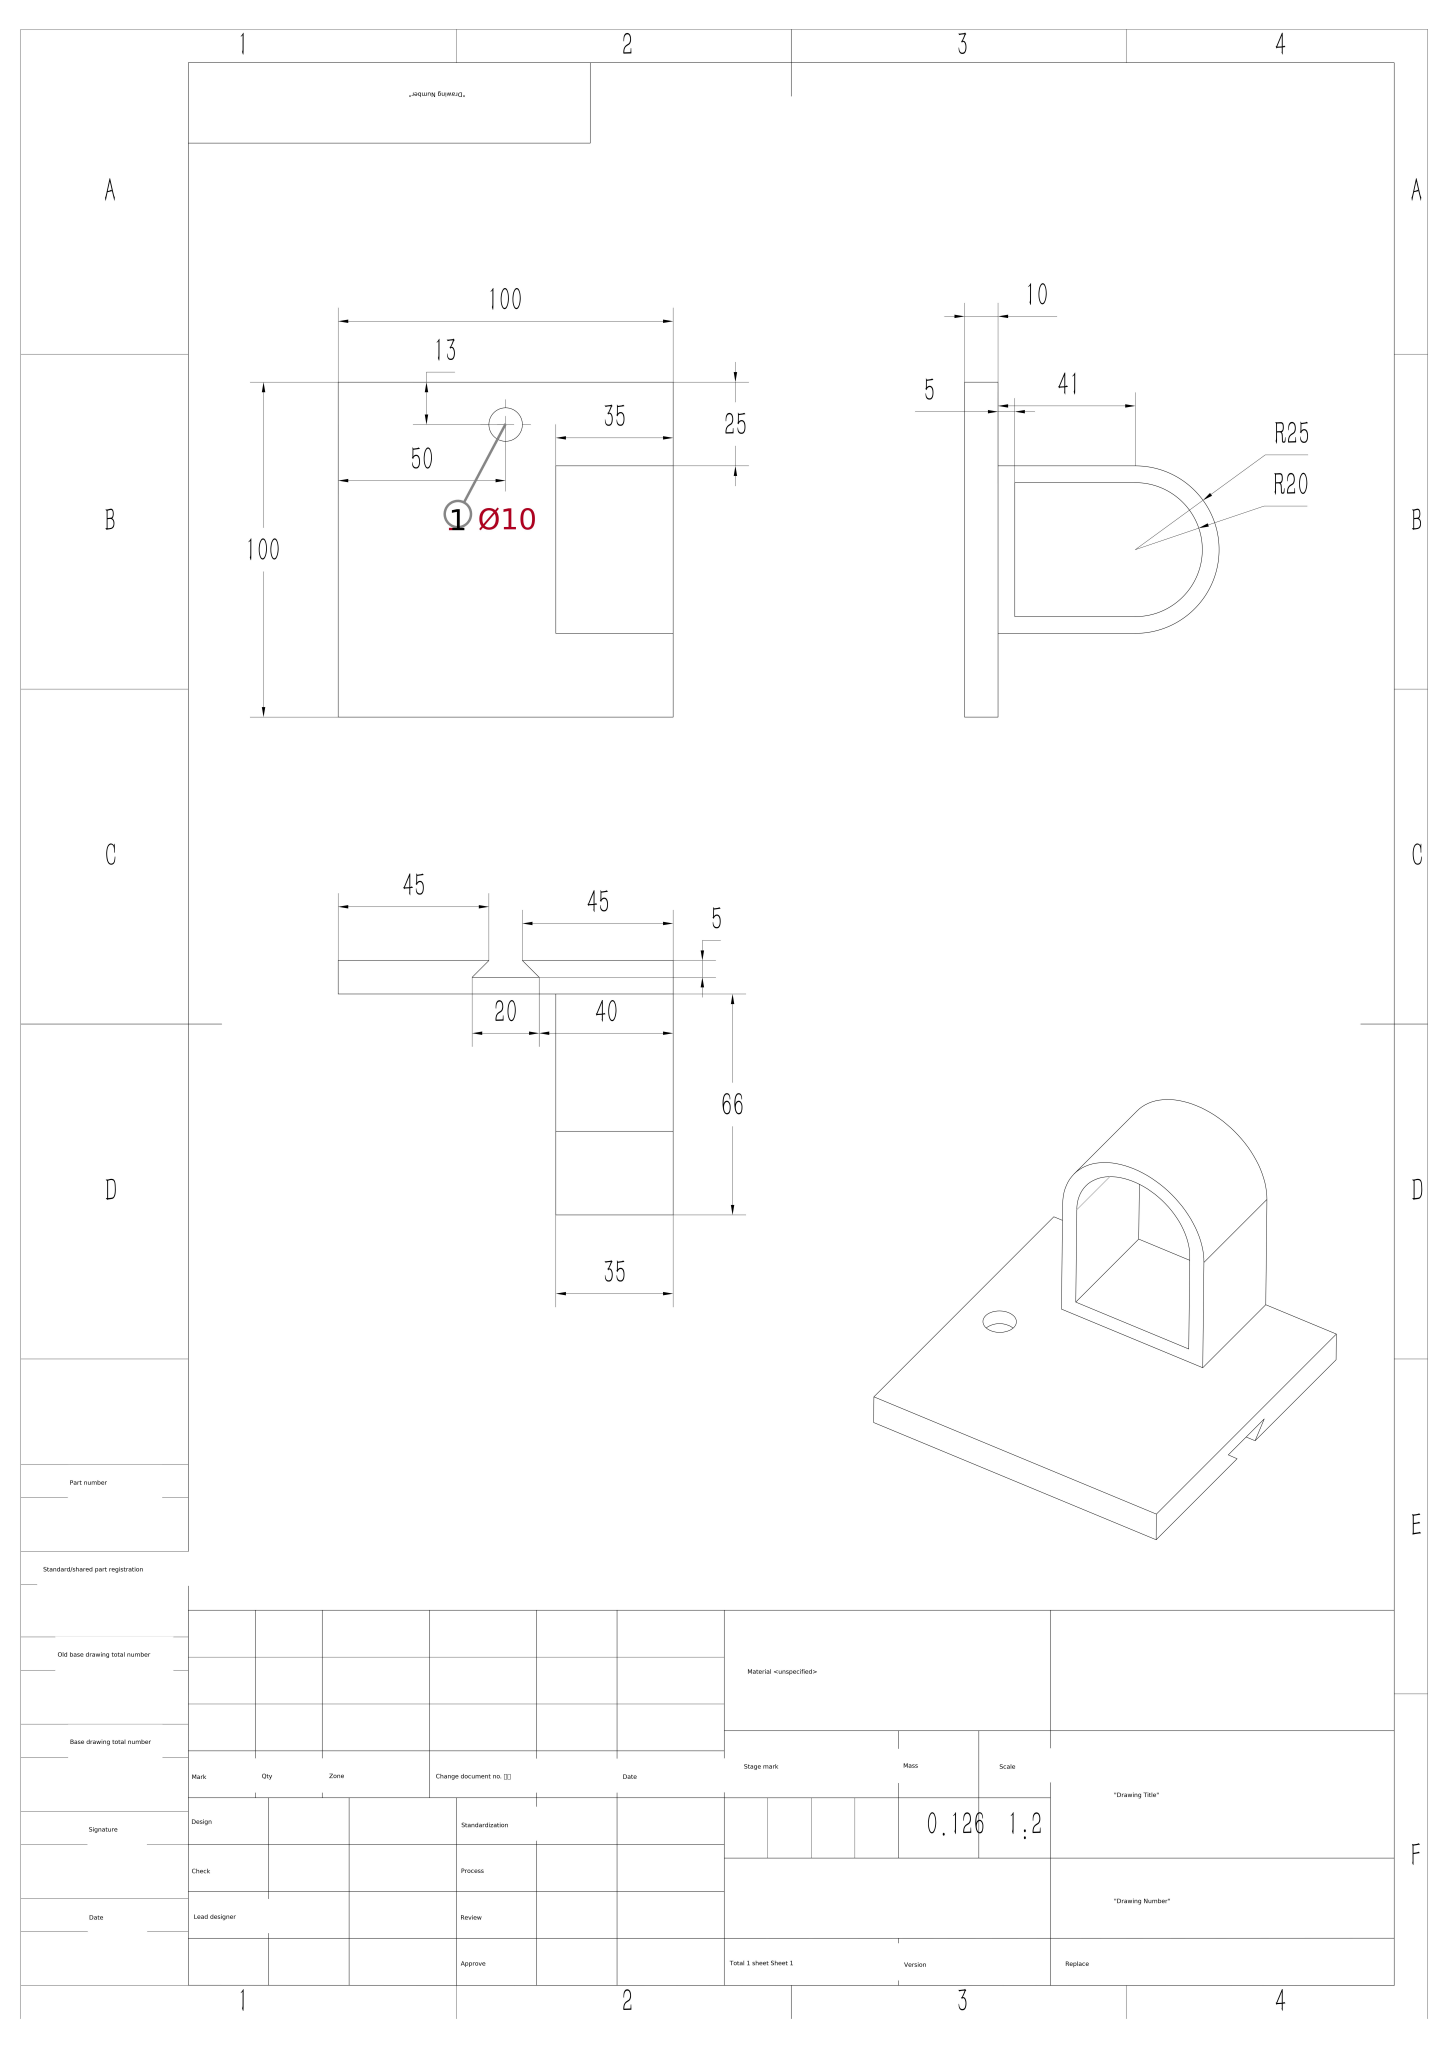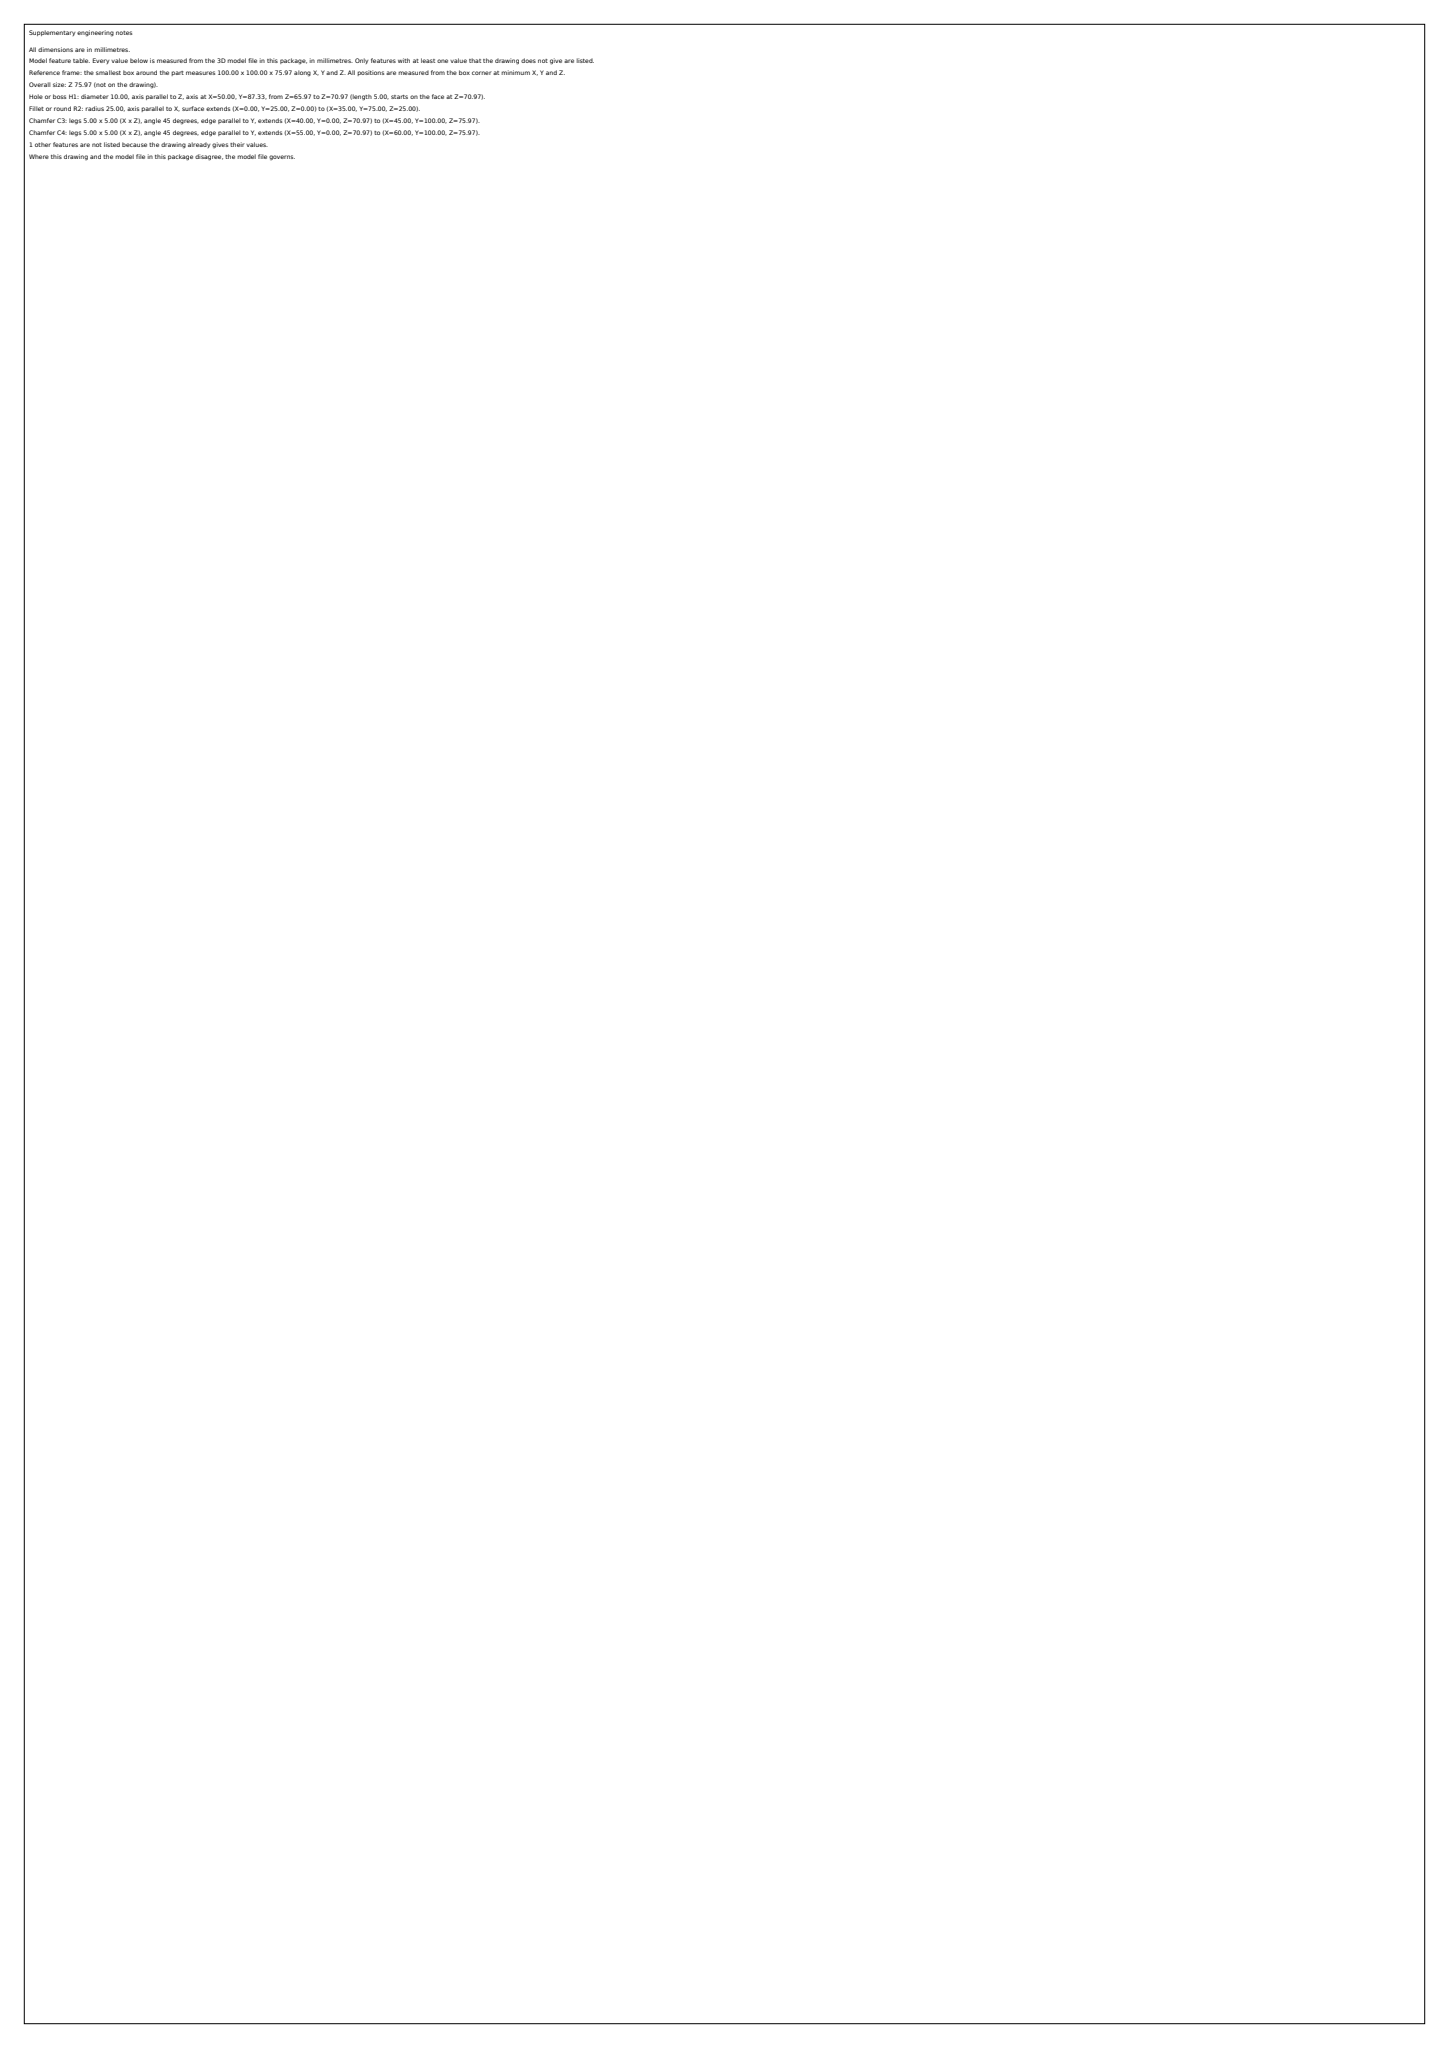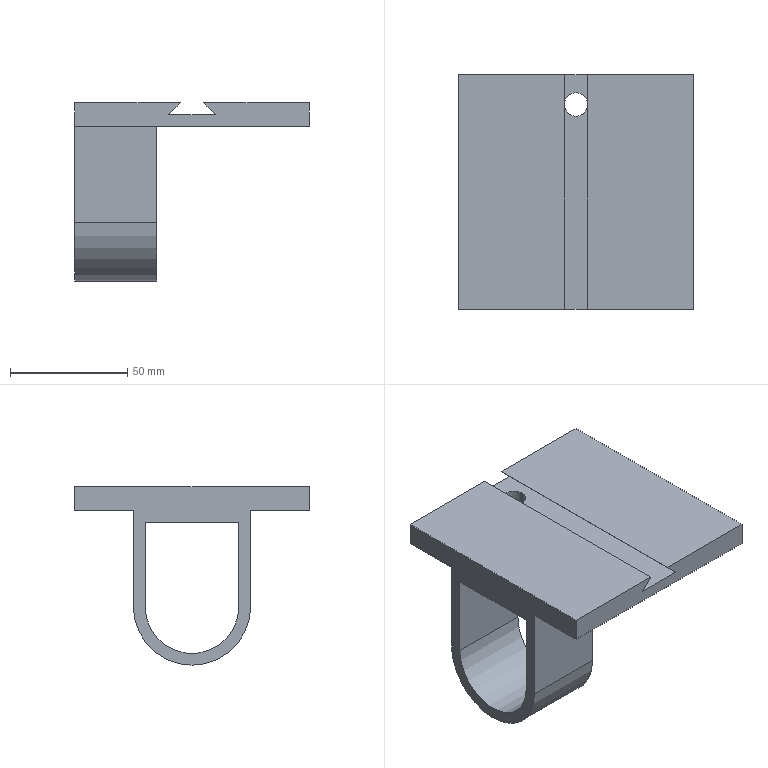Part | SolidWorks | mm | 1 solid | 20 faces | box 100 x 100 x 75.97 mm | volume 125816 mm3 | plane 16 | cylinder 4 | commonest cylinder face diameters 10 x2 50 x1 40 x1
build123d program:
from build123d import *

# Parameters (mm, degrees)
BOSS_EXTRUDE1_DEPTH = 100
SKETCH2_R           = 5
CUT_EXTRUDE1_DEPTH  = 113.25
BOSS_EXTRUDE2_DEPTH = 35


with BuildPart() as part:
    # Sketch1 → Boss-Extrude1 (new body)
    with BuildSketch(Plane(origin=(0, 0, 0), x_dir=(1, 0, 0), z_dir=(0, 1, 0))):
        Polygon((-50, -5), (-5, -5), (-10, 0), (10, 0), (5, -5), (50, -5), (50, 5), (-50, 5), align=None)
    extrude(amount=BOSS_EXTRUDE1_DEPTH)

    # Sketch2 → Cut-Extrude1 (cut, through all)
    with BuildSketch(Plane(origin=(0, 0, -5), x_dir=(-1, 0, 0), z_dir=(0, 0, -1))):
        with Locations((0, 87.33)):
            Circle(SKETCH2_R)
    extrude(amount=-CUT_EXTRUDE1_DEPTH, mode=Mode.SUBTRACT)

    # Sketch3 → Boss-Extrude2 (add)
    with BuildSketch(Plane.ZY.offset(50)):
        with BuildLine():
            Line((-5, 25), (-45.968, 25))
            ThreePointArc((-45.968, 25), (-70.968, 50), (-45.968, 75))
            Line((-45.968, 75), (-5, 75))
            Line((-5, 75), (-5, 70))
            Line((-5, 70), (-5, 30))
            Line((-5, 30), (-5, 25))
        make_face()
        with BuildLine():
            Line((-10, 30), (-45.968, 30))
            ThreePointArc((-45.968, 30), (-65.968, 50), (-45.968, 70))
            Line((-45.968, 70), (-10, 70))
            Line((-10, 70), (-10, 30))
        make_face(mode=Mode.SUBTRACT)
    extrude(amount=-BOSS_EXTRUDE2_DEPTH)


solid = part.part
STEP:
#1=CARTESIAN_POINT('',(5.,87.33,0.));
#2=VERTEX_POINT('',#1);
#3=CARTESIAN_POINT('',(-5.,87.33,0.));
#4=VERTEX_POINT('',#3);
#5=CARTESIAN_POINT('',(0.,87.33,0.));
#6=DIRECTION('',(0.,0.,-1.));
#7=DIRECTION('',(-1.,0.,0.));
#8=AXIS2_PLACEMENT_3D('',#5,#6,#7);
#9=CIRCLE('',#8,5.);
#10=EDGE_CURVE('',#2,#4,#9,.T.);
#11=ORIENTED_EDGE('',*,*,#10,.F.);
#12=CARTESIAN_POINT('',(5.,87.33,-5.));
#13=VERTEX_POINT('',#12);
#14=CARTESIAN_POINT('',(5.,87.33,5.));
#15=DIRECTION('',(0.,0.,-1.));
#16=VECTOR('',#15,1000.);
#17=LINE('',#14,#16);
#18=EDGE_CURVE('',#2,#13,#17,.T.);
#19=ORIENTED_EDGE('',*,*,#18,.T.);
#20=CARTESIAN_POINT('',(-5.,87.33,-5.));
#21=VERTEX_POINT('',#20);
#22=CARTESIAN_POINT('',(0.,87.33,-5.));
#23=DIRECTION('',(0.,0.,-1.));
#24=DIRECTION('',(-1.,0.,0.));
#25=AXIS2_PLACEMENT_3D('',#22,#23,#24);
#26=CIRCLE('',#25,5.);
#27=EDGE_CURVE('',#13,#21,#26,.T.);
#28=ORIENTED_EDGE('',*,*,#27,.T.);
#29=CARTESIAN_POINT('',(-5.,87.33,5.));
#30=DIRECTION('',(0.,0.,-1.));
#31=VECTOR('',#30,1000.);
#32=LINE('',#29,#31);
#33=EDGE_CURVE('',#4,#21,#32,.T.);
#34=ORIENTED_EDGE('',*,*,#33,.F.);
#35=EDGE_LOOP('',(#11,#19,#28,#34));
#36=FACE_OUTER_BOUND('',#35,.T.);
#37=CARTESIAN_POINT('',(0.,87.33,5.));
#38=DIRECTION('',(0.,0.,-1.));
#39=DIRECTION('',(-1.,0.,0.));
#40=AXIS2_PLACEMENT_3D('',#37,#38,#39);
#41=CYLINDRICAL_SURFACE('',#40,5.);
#42=ADVANCED_FACE('',(#36),#41,.F.);
#43=CARTESIAN_POINT('',(0.,87.33,-5.));
#44=DIRECTION('',(0.,0.,-1.));
#45=DIRECTION('',(-1.,0.,0.));
#46=AXIS2_PLACEMENT_3D('',#43,#44,#45);
#47=CIRCLE('',#46,5.);
#48=EDGE_CURVE('',#21,#13,#47,.T.);
#49=ORIENTED_EDGE('',*,*,#48,.F.);
#50=ORIENTED_EDGE('',*,*,#27,.F.);
#51=EDGE_LOOP('',(#49,#50));
#52=FACE_BOUND('',#51,.T.);
#53=CARTESIAN_POINT('',(-15.,25.,-5.));
#54=VERTEX_POINT('',#53);
#55=CARTESIAN_POINT('',(-50.,25.,-5.));
#56=VERTEX_POINT('',#55);
#57=CARTESIAN_POINT('',(-15.,25.,-5.));
#58=DIRECTION('',(-1.,0.,0.));
#59=VECTOR('',#58,1000.);
#60=LINE('',#57,#59);
#61=EDGE_CURVE('',#54,#56,#60,.T.);
#62=ORIENTED_EDGE('',*,*,#61,.F.);
#63=CARTESIAN_POINT('',(-15.,75.,-5.));
#64=VERTEX_POINT('',#63);
#65=CARTESIAN_POINT('',(-15.,30.,-5.));
#66=DIRECTION('',(0.,1.,-0.));
#67=VECTOR('',#66,1000.);
#68=LINE('',#65,#67);
#69=EDGE_CURVE('',#54,#64,#68,.T.);
#70=ORIENTED_EDGE('',*,*,#69,.T.);
#71=CARTESIAN_POINT('',(-50.,75.,-5.));
#72=VERTEX_POINT('',#71);
#73=CARTESIAN_POINT('',(-15.,75.,-5.));
#74=DIRECTION('',(-1.,0.,0.));
#75=VECTOR('',#74,1000.);
#76=LINE('',#73,#75);
#77=EDGE_CURVE('',#64,#72,#76,.T.);
#78=ORIENTED_EDGE('',*,*,#77,.T.);
#79=CARTESIAN_POINT('',(-50.,100.,-5.));
#80=VERTEX_POINT('',#79);
#81=CARTESIAN_POINT('',(-50.,100.,-5.));
#82=DIRECTION('',(0.,-1.,0.));
#83=VECTOR('',#82,1000.);
#84=LINE('',#81,#83);
#85=EDGE_CURVE('',#80,#72,#84,.T.);
#86=ORIENTED_EDGE('',*,*,#85,.F.);
#87=CARTESIAN_POINT('',(50.,100.,-5.));
#88=VERTEX_POINT('',#87);
#89=CARTESIAN_POINT('',(-50.,100.,-5.));
#90=DIRECTION('',(-1.,0.,0.));
#91=VECTOR('',#90,1000.);
#92=LINE('',#89,#91);
#93=EDGE_CURVE('',#88,#80,#92,.T.);
#94=ORIENTED_EDGE('',*,*,#93,.F.);
#95=CARTESIAN_POINT('',(50.,0.,-5.));
#96=VERTEX_POINT('',#95);
#97=CARTESIAN_POINT('',(50.,100.,-5.));
#98=DIRECTION('',(0.,-1.,0.));
#99=VECTOR('',#98,1000.);
#100=LINE('',#97,#99);
#101=EDGE_CURVE('',#88,#96,#100,.T.);
#102=ORIENTED_EDGE('',*,*,#101,.T.);
#103=CARTESIAN_POINT('',(-50.,0.,-5.));
#104=VERTEX_POINT('',#103);
#105=CARTESIAN_POINT('',(-50.,0.,-5.));
#106=DIRECTION('',(-1.,0.,0.));
#107=VECTOR('',#106,1000.);
#108=LINE('',#105,#107);
#109=EDGE_CURVE('',#96,#104,#108,.T.);
#110=ORIENTED_EDGE('',*,*,#109,.T.);
#111=CARTESIAN_POINT('',(-50.,100.,-5.));
#112=DIRECTION('',(0.,-1.,0.));
#113=VECTOR('',#112,1000.);
#114=LINE('',#111,#113);
#115=EDGE_CURVE('',#56,#104,#114,.T.);
#116=ORIENTED_EDGE('',*,*,#115,.F.);
#117=EDGE_LOOP('',(#62,#70,#78,#86,#94,#102,#110,#116));
#118=FACE_OUTER_BOUND('',#117,.T.);
#119=CARTESIAN_POINT('',(-50.,100.,-5.));
#120=DIRECTION('',(0.,0.,1.));
#121=DIRECTION('',(1.,0.,0.));
#122=AXIS2_PLACEMENT_3D('',#119,#120,#121);
#123=PLANE('',#122);
#124=ADVANCED_FACE('',(#52,#118),#123,.F.);
#125=CARTESIAN_POINT('',(50.,0.,5.));
#126=VERTEX_POINT('',#125);
#127=CARTESIAN_POINT('',(50.,0.,5.));
#128=DIRECTION('',(0.,0.,-1.));
#129=VECTOR('',#128,1000.);
#130=LINE('',#127,#129);
#131=EDGE_CURVE('',#126,#96,#130,.T.);
#132=ORIENTED_EDGE('',*,*,#131,.T.);
#133=ORIENTED_EDGE('',*,*,#101,.F.);
#134=CARTESIAN_POINT('',(50.,100.,5.));
#135=VERTEX_POINT('',#134);
#136=CARTESIAN_POINT('',(50.,100.,5.));
#137=DIRECTION('',(0.,0.,-1.));
#138=VECTOR('',#137,1000.);
#139=LINE('',#136,#138);
#140=EDGE_CURVE('',#135,#88,#139,.T.);
#141=ORIENTED_EDGE('',*,*,#140,.F.);
#142=CARTESIAN_POINT('',(50.,100.,5.));
#143=DIRECTION('',(0.,-1.,0.));
#144=VECTOR('',#143,1000.);
#145=LINE('',#142,#144);
#146=EDGE_CURVE('',#135,#126,#145,.T.);
#147=ORIENTED_EDGE('',*,*,#146,.T.);
#148=EDGE_LOOP('',(#132,#133,#141,#147));
#149=FACE_OUTER_BOUND('',#148,.T.);
#150=CARTESIAN_POINT('',(50.,100.,5.));
#151=DIRECTION('',(-1.,0.,0.));
#152=DIRECTION('',(0.,0.,1.));
#153=AXIS2_PLACEMENT_3D('',#150,#151,#152);
#154=PLANE('',#153);
#155=ADVANCED_FACE('',(#149),#154,.F.);
#156=CARTESIAN_POINT('',(-50.,0.,5.));
#157=VERTEX_POINT('',#156);
#158=CARTESIAN_POINT('',(-50.,0.,5.));
#159=DIRECTION('',(0.,0.,1.));
#160=VECTOR('',#159,1000.);
#161=LINE('',#158,#160);
#162=EDGE_CURVE('',#104,#157,#161,.T.);
#163=ORIENTED_EDGE('',*,*,#162,.T.);
#164=CARTESIAN_POINT('',(-50.,100.,5.));
#165=VERTEX_POINT('',#164);
#166=CARTESIAN_POINT('',(-50.,100.,5.));
#167=DIRECTION('',(0.,-1.,0.));
#168=VECTOR('',#167,1000.);
#169=LINE('',#166,#168);
#170=EDGE_CURVE('',#165,#157,#169,.T.);
#171=ORIENTED_EDGE('',*,*,#170,.F.);
#172=CARTESIAN_POINT('',(-50.,100.,5.));
#173=DIRECTION('',(0.,0.,1.));
#174=VECTOR('',#173,1000.);
#175=LINE('',#172,#174);
#176=EDGE_CURVE('',#80,#165,#175,.T.);
#177=ORIENTED_EDGE('',*,*,#176,.F.);
#178=ORIENTED_EDGE('',*,*,#85,.T.);
#179=CARTESIAN_POINT('',(-50.,75.,-45.968));
#180=VERTEX_POINT('',#179);
#181=CARTESIAN_POINT('',(-50.,75.,-5.));
#182=DIRECTION('',(0.,-0.,-1.));
#183=VECTOR('',#182,1000.);
#184=LINE('',#181,#183);
#185=EDGE_CURVE('',#72,#180,#184,.T.);
#186=ORIENTED_EDGE('',*,*,#185,.T.);
#187=CARTESIAN_POINT('',(-50.,25.,-45.968));
#188=VERTEX_POINT('',#187);
#189=CARTESIAN_POINT('',(-50.,50.,-45.968));
#190=DIRECTION('',(-1.,0.,0.));
#191=DIRECTION('',(0.,0.,1.));
#192=AXIS2_PLACEMENT_3D('',#189,#190,#191);
#193=CIRCLE('',#192,25.);
#194=EDGE_CURVE('',#180,#188,#193,.T.);
#195=ORIENTED_EDGE('',*,*,#194,.T.);
#196=CARTESIAN_POINT('',(-50.,25.,-5.));
#197=DIRECTION('',(0.,0.,1.));
#198=VECTOR('',#197,1000.);
#199=LINE('',#196,#198);
#200=EDGE_CURVE('',#188,#56,#199,.T.);
#201=ORIENTED_EDGE('',*,*,#200,.T.);
#202=ORIENTED_EDGE('',*,*,#115,.T.);
#203=EDGE_LOOP('',(#163,#171,#177,#178,#186,#195,#201,#202));
#204=FACE_OUTER_BOUND('',#203,.T.);
#205=CARTESIAN_POINT('',(-50.,70.,-45.968));
#206=VERTEX_POINT('',#205);
#207=CARTESIAN_POINT('',(-50.,30.,-45.968));
#208=VERTEX_POINT('',#207);
#209=CARTESIAN_POINT('',(-50.,50.,-45.968));
#210=DIRECTION('',(-1.,0.,0.));
#211=DIRECTION('',(0.,0.,1.));
#212=AXIS2_PLACEMENT_3D('',#209,#210,#211);
#213=CIRCLE('',#212,20.);
#214=EDGE_CURVE('',#206,#208,#213,.T.);
#215=ORIENTED_EDGE('',*,*,#214,.F.);
#216=CARTESIAN_POINT('',(-50.,70.,-10.));
#217=VERTEX_POINT('',#216);
#218=CARTESIAN_POINT('',(-50.,70.,-10.));
#219=DIRECTION('',(0.,0.,-1.));
#220=VECTOR('',#219,1000.);
#221=LINE('',#218,#220);
#222=EDGE_CURVE('',#217,#206,#221,.T.);
#223=ORIENTED_EDGE('',*,*,#222,.F.);
#224=CARTESIAN_POINT('',(-50.,30.,-10.));
#225=VERTEX_POINT('',#224);
#226=CARTESIAN_POINT('',(-50.,70.,-10.));
#227=DIRECTION('',(0.,1.,-0.));
#228=VECTOR('',#227,1000.);
#229=LINE('',#226,#228);
#230=EDGE_CURVE('',#225,#217,#229,.T.);
#231=ORIENTED_EDGE('',*,*,#230,.F.);
#232=CARTESIAN_POINT('',(-50.,30.,-10.));
#233=DIRECTION('',(0.,0.,1.));
#234=VECTOR('',#233,1000.);
#235=LINE('',#232,#234);
#236=EDGE_CURVE('',#208,#225,#235,.T.);
#237=ORIENTED_EDGE('',*,*,#236,.F.);
#238=EDGE_LOOP('',(#215,#223,#231,#237));
#239=FACE_BOUND('',#238,.T.);
#240=CARTESIAN_POINT('',(-50.,100.,5.));
#241=DIRECTION('',(1.,0.,0.));
#242=DIRECTION('',(0.,0.,-1.));
#243=AXIS2_PLACEMENT_3D('',#240,#241,#242);
#244=PLANE('',#243);
#245=ADVANCED_FACE('',(#204,#239),#244,.F.);
#246=CARTESIAN_POINT('',(-5.,0.,5.));
#247=VERTEX_POINT('',#246);
#248=CARTESIAN_POINT('',(-50.,0.,5.));
#249=DIRECTION('',(1.,0.,0.));
#250=VECTOR('',#249,1000.);
#251=LINE('',#248,#250);
#252=EDGE_CURVE('',#157,#247,#251,.T.);
#253=ORIENTED_EDGE('',*,*,#252,.T.);
#254=CARTESIAN_POINT('',(-5.,100.,5.));
#255=VERTEX_POINT('',#254);
#256=CARTESIAN_POINT('',(-5.,100.,5.));
#257=DIRECTION('',(0.,-1.,0.));
#258=VECTOR('',#257,1000.);
#259=LINE('',#256,#258);
#260=EDGE_CURVE('',#255,#247,#259,.T.);
#261=ORIENTED_EDGE('',*,*,#260,.F.);
#262=CARTESIAN_POINT('',(-50.,100.,5.));
#263=DIRECTION('',(1.,0.,0.));
#264=VECTOR('',#263,1000.);
#265=LINE('',#262,#264);
#266=EDGE_CURVE('',#165,#255,#265,.T.);
#267=ORIENTED_EDGE('',*,*,#266,.F.);
#268=ORIENTED_EDGE('',*,*,#170,.T.);
#269=EDGE_LOOP('',(#253,#261,#267,#268));
#270=FACE_OUTER_BOUND('',#269,.T.);
#271=CARTESIAN_POINT('',(-50.,100.,5.));
#272=DIRECTION('',(0.,0.,-1.));
#273=DIRECTION('',(-1.,0.,0.));
#274=AXIS2_PLACEMENT_3D('',#271,#272,#273);
#275=PLANE('',#274);
#276=ADVANCED_FACE('',(#270),#275,.F.);
#277=CARTESIAN_POINT('',(-10.,0.,0.));
#278=VERTEX_POINT('',#277);
#279=CARTESIAN_POINT('',(-5.,0.,5.));
#280=DIRECTION('',(-0.7071,0.,-0.7071));
#281=VECTOR('',#280,1000.);
#282=LINE('',#279,#281);
#283=EDGE_CURVE('',#247,#278,#282,.T.);
#284=ORIENTED_EDGE('',*,*,#283,.T.);
#285=CARTESIAN_POINT('',(-10.,100.,0.));
#286=VERTEX_POINT('',#285);
#287=CARTESIAN_POINT('',(-10.,100.,0.));
#288=DIRECTION('',(0.,-1.,0.));
#289=VECTOR('',#288,1000.);
#290=LINE('',#287,#289);
#291=EDGE_CURVE('',#286,#278,#290,.T.);
#292=ORIENTED_EDGE('',*,*,#291,.F.);
#293=CARTESIAN_POINT('',(-5.,100.,5.));
#294=DIRECTION('',(-0.7071,0.,-0.7071));
#295=VECTOR('',#294,1000.);
#296=LINE('',#293,#295);
#297=EDGE_CURVE('',#255,#286,#296,.T.);
#298=ORIENTED_EDGE('',*,*,#297,.F.);
#299=ORIENTED_EDGE('',*,*,#260,.T.);
#300=EDGE_LOOP('',(#284,#292,#298,#299));
#301=FACE_OUTER_BOUND('',#300,.T.);
#302=CARTESIAN_POINT('',(-5.,100.,5.));
#303=DIRECTION('',(-0.7071,0.,0.7071));
#304=DIRECTION('',(0.7071,0.,0.7071));
#305=AXIS2_PLACEMENT_3D('',#302,#303,#304);
#306=PLANE('',#305);
#307=ADVANCED_FACE('',(#301),#306,.F.);
#308=CARTESIAN_POINT('',(0.,87.33,0.));
#309=DIRECTION('',(0.,0.,-1.));
#310=DIRECTION('',(-1.,0.,0.));
#311=AXIS2_PLACEMENT_3D('',#308,#309,#310);
#312=CIRCLE('',#311,5.);
#313=EDGE_CURVE('',#4,#2,#312,.T.);
#314=ORIENTED_EDGE('',*,*,#313,.T.);
#315=ORIENTED_EDGE('',*,*,#10,.T.);
#316=EDGE_LOOP('',(#314,#315));
#317=FACE_BOUND('',#316,.T.);
#318=CARTESIAN_POINT('',(10.,0.,0.));
#319=VERTEX_POINT('',#318);
#320=CARTESIAN_POINT('',(-10.,0.,0.));
#321=DIRECTION('',(1.,0.,0.));
#322=VECTOR('',#321,1000.);
#323=LINE('',#320,#322);
#324=EDGE_CURVE('',#278,#319,#323,.T.);
#325=ORIENTED_EDGE('',*,*,#324,.T.);
#326=CARTESIAN_POINT('',(10.,100.,0.));
#327=VERTEX_POINT('',#326);
#328=CARTESIAN_POINT('',(10.,100.,0.));
#329=DIRECTION('',(0.,-1.,0.));
#330=VECTOR('',#329,1000.);
#331=LINE('',#328,#330);
#332=EDGE_CURVE('',#327,#319,#331,.T.);
#333=ORIENTED_EDGE('',*,*,#332,.F.);
#334=CARTESIAN_POINT('',(-10.,100.,0.));
#335=DIRECTION('',(1.,0.,0.));
#336=VECTOR('',#335,1000.);
#337=LINE('',#334,#336);
#338=EDGE_CURVE('',#286,#327,#337,.T.);
#339=ORIENTED_EDGE('',*,*,#338,.F.);
#340=ORIENTED_EDGE('',*,*,#291,.T.);
#341=EDGE_LOOP('',(#325,#333,#339,#340));
#342=FACE_OUTER_BOUND('',#341,.T.);
#343=CARTESIAN_POINT('',(-10.,100.,0.));
#344=DIRECTION('',(0.,0.,-1.));
#345=DIRECTION('',(-1.,0.,0.));
#346=AXIS2_PLACEMENT_3D('',#343,#344,#345);
#347=PLANE('',#346);
#348=ADVANCED_FACE('',(#317,#342),#347,.F.);
#349=CARTESIAN_POINT('',(5.,0.,5.));
#350=VERTEX_POINT('',#349);
#351=CARTESIAN_POINT('',(10.,0.,0.));
#352=DIRECTION('',(-0.7071,0.,0.7071));
#353=VECTOR('',#352,1000.);
#354=LINE('',#351,#353);
#355=EDGE_CURVE('',#319,#350,#354,.T.);
#356=ORIENTED_EDGE('',*,*,#355,.T.);
#357=CARTESIAN_POINT('',(5.,100.,5.));
#358=VERTEX_POINT('',#357);
#359=CARTESIAN_POINT('',(5.,100.,5.));
#360=DIRECTION('',(0.,-1.,0.));
#361=VECTOR('',#360,1000.);
#362=LINE('',#359,#361);
#363=EDGE_CURVE('',#358,#350,#362,.T.);
#364=ORIENTED_EDGE('',*,*,#363,.F.);
#365=CARTESIAN_POINT('',(10.,100.,0.));
#366=DIRECTION('',(-0.7071,0.,0.7071));
#367=VECTOR('',#366,1000.);
#368=LINE('',#365,#367);
#369=EDGE_CURVE('',#327,#358,#368,.T.);
#370=ORIENTED_EDGE('',*,*,#369,.F.);
#371=ORIENTED_EDGE('',*,*,#332,.T.);
#372=EDGE_LOOP('',(#356,#364,#370,#371));
#373=FACE_OUTER_BOUND('',#372,.T.);
#374=CARTESIAN_POINT('',(10.,100.,0.));
#375=DIRECTION('',(0.7071,0.,0.7071));
#376=DIRECTION('',(0.7071,0.,-0.7071));
#377=AXIS2_PLACEMENT_3D('',#374,#375,#376);
#378=PLANE('',#377);
#379=ADVANCED_FACE('',(#373),#378,.F.);
#380=CARTESIAN_POINT('',(5.,0.,5.));
#381=DIRECTION('',(1.,0.,0.));
#382=VECTOR('',#381,1000.);
#383=LINE('',#380,#382);
#384=EDGE_CURVE('',#350,#126,#383,.T.);
#385=ORIENTED_EDGE('',*,*,#384,.T.);
#386=ORIENTED_EDGE('',*,*,#146,.F.);
#387=CARTESIAN_POINT('',(5.,100.,5.));
#388=DIRECTION('',(1.,0.,0.));
#389=VECTOR('',#388,1000.);
#390=LINE('',#387,#389);
#391=EDGE_CURVE('',#358,#135,#390,.T.);
#392=ORIENTED_EDGE('',*,*,#391,.F.);
#393=ORIENTED_EDGE('',*,*,#363,.T.);
#394=EDGE_LOOP('',(#385,#386,#392,#393));
#395=FACE_OUTER_BOUND('',#394,.T.);
#396=CARTESIAN_POINT('',(5.,100.,5.));
#397=DIRECTION('',(0.,0.,-1.));
#398=DIRECTION('',(-1.,0.,0.));
#399=AXIS2_PLACEMENT_3D('',#396,#397,#398);
#400=PLANE('',#399);
#401=ADVANCED_FACE('',(#395),#400,.F.);
#402=ORIENTED_EDGE('',*,*,#140,.T.);
#403=ORIENTED_EDGE('',*,*,#93,.T.);
#404=ORIENTED_EDGE('',*,*,#176,.T.);
#405=ORIENTED_EDGE('',*,*,#266,.T.);
#406=ORIENTED_EDGE('',*,*,#297,.T.);
#407=ORIENTED_EDGE('',*,*,#338,.T.);
#408=ORIENTED_EDGE('',*,*,#369,.T.);
#409=ORIENTED_EDGE('',*,*,#391,.T.);
#410=EDGE_LOOP('',(#402,#403,#404,#405,#406,#407,#408,#409));
#411=FACE_OUTER_BOUND('',#410,.T.);
#412=CARTESIAN_POINT('',(0.,100.,0.));
#413=DIRECTION('',(0.,-1.,0.));
#414=DIRECTION('',(0.,0.,-1.));
#415=AXIS2_PLACEMENT_3D('',#412,#413,#414);
#416=PLANE('',#415);
#417=ADVANCED_FACE('',(#411),#416,.F.);
#418=ORIENTED_EDGE('',*,*,#131,.F.);
#419=ORIENTED_EDGE('',*,*,#384,.F.);
#420=ORIENTED_EDGE('',*,*,#355,.F.);
#421=ORIENTED_EDGE('',*,*,#324,.F.);
#422=ORIENTED_EDGE('',*,*,#283,.F.);
#423=ORIENTED_EDGE('',*,*,#252,.F.);
#424=ORIENTED_EDGE('',*,*,#162,.F.);
#425=ORIENTED_EDGE('',*,*,#109,.F.);
#426=EDGE_LOOP('',(#418,#419,#420,#421,#422,#423,#424,#425));
#427=FACE_OUTER_BOUND('',#426,.T.);
#428=CARTESIAN_POINT('',(0.,0.,0.));
#429=DIRECTION('',(0.,-1.,0.));
#430=DIRECTION('',(0.,0.,-1.));
#431=AXIS2_PLACEMENT_3D('',#428,#429,#430);
#432=PLANE('',#431);
#433=ADVANCED_FACE('',(#427),#432,.T.);
#434=ORIENTED_EDGE('',*,*,#18,.F.);
#435=ORIENTED_EDGE('',*,*,#313,.F.);
#436=ORIENTED_EDGE('',*,*,#33,.T.);
#437=ORIENTED_EDGE('',*,*,#48,.T.);
#438=EDGE_LOOP('',(#434,#435,#436,#437));
#439=FACE_OUTER_BOUND('',#438,.T.);
#440=CARTESIAN_POINT('',(0.,87.33,5.));
#441=DIRECTION('',(0.,0.,-1.));
#442=DIRECTION('',(-1.,0.,0.));
#443=AXIS2_PLACEMENT_3D('',#440,#441,#442);
#444=CYLINDRICAL_SURFACE('',#443,5.);
#445=ADVANCED_FACE('',(#439),#444,.F.);
#446=ORIENTED_EDGE('',*,*,#200,.F.);
#447=CARTESIAN_POINT('',(-15.,25.,-45.968));
#448=VERTEX_POINT('',#447);
#449=CARTESIAN_POINT('',(-15.,25.,-45.968));
#450=DIRECTION('',(-1.,0.,0.));
#451=VECTOR('',#450,1000.);
#452=LINE('',#449,#451);
#453=EDGE_CURVE('',#448,#188,#452,.T.);
#454=ORIENTED_EDGE('',*,*,#453,.F.);
#455=CARTESIAN_POINT('',(-15.,25.,-5.));
#456=DIRECTION('',(0.,0.,1.));
#457=VECTOR('',#456,1000.);
#458=LINE('',#455,#457);
#459=EDGE_CURVE('',#448,#54,#458,.T.);
#460=ORIENTED_EDGE('',*,*,#459,.T.);
#461=ORIENTED_EDGE('',*,*,#61,.T.);
#462=EDGE_LOOP('',(#446,#454,#460,#461));
#463=FACE_OUTER_BOUND('',#462,.T.);
#464=CARTESIAN_POINT('',(-15.,25.,-5.));
#465=DIRECTION('',(0.,-1.,0.));
#466=DIRECTION('',(0.,-0.,-1.));
#467=AXIS2_PLACEMENT_3D('',#464,#465,#466);
#468=PLANE('',#467);
#469=ADVANCED_FACE('',(#463),#468,.T.);
#470=ORIENTED_EDGE('',*,*,#194,.F.);
#471=CARTESIAN_POINT('',(-15.,75.,-45.968));
#472=VERTEX_POINT('',#471);
#473=CARTESIAN_POINT('',(-15.,75.,-45.968));
#474=DIRECTION('',(-1.,0.,0.));
#475=VECTOR('',#474,1000.);
#476=LINE('',#473,#475);
#477=EDGE_CURVE('',#472,#180,#476,.T.);
#478=ORIENTED_EDGE('',*,*,#477,.F.);
#479=CARTESIAN_POINT('',(-15.,50.,-45.968));
#480=DIRECTION('',(-1.,0.,0.));
#481=DIRECTION('',(0.,0.,1.));
#482=AXIS2_PLACEMENT_3D('',#479,#480,#481);
#483=CIRCLE('',#482,25.);
#484=EDGE_CURVE('',#472,#448,#483,.T.);
#485=ORIENTED_EDGE('',*,*,#484,.T.);
#486=ORIENTED_EDGE('',*,*,#453,.T.);
#487=EDGE_LOOP('',(#470,#478,#485,#486));
#488=FACE_OUTER_BOUND('',#487,.T.);
#489=CARTESIAN_POINT('',(-15.,50.,-45.968));
#490=DIRECTION('',(-1.,0.,0.));
#491=DIRECTION('',(0.,0.,1.));
#492=AXIS2_PLACEMENT_3D('',#489,#490,#491);
#493=CYLINDRICAL_SURFACE('',#492,25.);
#494=ADVANCED_FACE('',(#488),#493,.T.);
#495=ORIENTED_EDGE('',*,*,#185,.F.);
#496=ORIENTED_EDGE('',*,*,#77,.F.);
#497=CARTESIAN_POINT('',(-15.,75.,-5.));
#498=DIRECTION('',(0.,-0.,-1.));
#499=VECTOR('',#498,1000.);
#500=LINE('',#497,#499);
#501=EDGE_CURVE('',#64,#472,#500,.T.);
#502=ORIENTED_EDGE('',*,*,#501,.T.);
#503=ORIENTED_EDGE('',*,*,#477,.T.);
#504=EDGE_LOOP('',(#495,#496,#502,#503));
#505=FACE_OUTER_BOUND('',#504,.T.);
#506=CARTESIAN_POINT('',(-15.,75.,-5.));
#507=DIRECTION('',(0.,1.,-0.));
#508=DIRECTION('',(0.,0.,1.));
#509=AXIS2_PLACEMENT_3D('',#506,#507,#508);
#510=PLANE('',#509);
#511=ADVANCED_FACE('',(#505),#510,.T.);
#512=CARTESIAN_POINT('',(-15.,70.,-10.));
#513=VERTEX_POINT('',#512);
#514=CARTESIAN_POINT('',(-15.,70.,-45.968));
#515=VERTEX_POINT('',#514);
#516=CARTESIAN_POINT('',(-15.,70.,-10.));
#517=DIRECTION('',(0.,0.,-1.));
#518=VECTOR('',#517,1000.);
#519=LINE('',#516,#518);
#520=EDGE_CURVE('',#513,#515,#519,.T.);
#521=ORIENTED_EDGE('',*,*,#520,.T.);
#522=CARTESIAN_POINT('',(-15.,30.,-45.968));
#523=VERTEX_POINT('',#522);
#524=CARTESIAN_POINT('',(-15.,50.,-45.968));
#525=DIRECTION('',(-1.,0.,0.));
#526=DIRECTION('',(0.,0.,1.));
#527=AXIS2_PLACEMENT_3D('',#524,#525,#526);
#528=CIRCLE('',#527,20.);
#529=EDGE_CURVE('',#515,#523,#528,.T.);
#530=ORIENTED_EDGE('',*,*,#529,.T.);
#531=CARTESIAN_POINT('',(-15.,30.,-10.));
#532=VERTEX_POINT('',#531);
#533=CARTESIAN_POINT('',(-15.,30.,-10.));
#534=DIRECTION('',(0.,0.,1.));
#535=VECTOR('',#534,1000.);
#536=LINE('',#533,#535);
#537=EDGE_CURVE('',#523,#532,#536,.T.);
#538=ORIENTED_EDGE('',*,*,#537,.T.);
#539=CARTESIAN_POINT('',(-15.,70.,-10.));
#540=DIRECTION('',(0.,1.,-0.));
#541=VECTOR('',#540,1000.);
#542=LINE('',#539,#541);
#543=EDGE_CURVE('',#532,#513,#542,.T.);
#544=ORIENTED_EDGE('',*,*,#543,.T.);
#545=EDGE_LOOP('',(#521,#530,#538,#544));
#546=FACE_BOUND('',#545,.T.);
#547=ORIENTED_EDGE('',*,*,#69,.F.);
#548=ORIENTED_EDGE('',*,*,#459,.F.);
#549=ORIENTED_EDGE('',*,*,#484,.F.);
#550=ORIENTED_EDGE('',*,*,#501,.F.);
#551=EDGE_LOOP('',(#547,#548,#549,#550));
#552=FACE_OUTER_BOUND('',#551,.T.);
#553=CARTESIAN_POINT('',(-15.,50.,-45.968));
#554=DIRECTION('',(-1.,0.,0.));
#555=DIRECTION('',(0.,0.,1.));
#556=AXIS2_PLACEMENT_3D('',#553,#554,#555);
#557=PLANE('',#556);
#558=ADVANCED_FACE('',(#546,#552),#557,.F.);
#559=ORIENTED_EDGE('',*,*,#214,.T.);
#560=CARTESIAN_POINT('',(-15.,30.,-45.968));
#561=DIRECTION('',(-1.,0.,0.));
#562=VECTOR('',#561,1000.);
#563=LINE('',#560,#562);
#564=EDGE_CURVE('',#523,#208,#563,.T.);
#565=ORIENTED_EDGE('',*,*,#564,.F.);
#566=ORIENTED_EDGE('',*,*,#529,.F.);
#567=CARTESIAN_POINT('',(-15.,70.,-45.968));
#568=DIRECTION('',(-1.,0.,0.));
#569=VECTOR('',#568,1000.);
#570=LINE('',#567,#569);
#571=EDGE_CURVE('',#515,#206,#570,.T.);
#572=ORIENTED_EDGE('',*,*,#571,.T.);
#573=EDGE_LOOP('',(#559,#565,#566,#572));
#574=FACE_OUTER_BOUND('',#573,.T.);
#575=CARTESIAN_POINT('',(-15.,50.,-45.968));
#576=DIRECTION('',(-1.,0.,0.));
#577=DIRECTION('',(0.,0.,1.));
#578=AXIS2_PLACEMENT_3D('',#575,#576,#577);
#579=CYLINDRICAL_SURFACE('',#578,20.);
#580=ADVANCED_FACE('',(#574),#579,.F.);
#581=ORIENTED_EDGE('',*,*,#222,.T.);
#582=ORIENTED_EDGE('',*,*,#571,.F.);
#583=ORIENTED_EDGE('',*,*,#520,.F.);
#584=CARTESIAN_POINT('',(-15.,70.,-10.));
#585=DIRECTION('',(-1.,0.,0.));
#586=VECTOR('',#585,1000.);
#587=LINE('',#584,#586);
#588=EDGE_CURVE('',#513,#217,#587,.T.);
#589=ORIENTED_EDGE('',*,*,#588,.T.);
#590=EDGE_LOOP('',(#581,#582,#583,#589));
#591=FACE_OUTER_BOUND('',#590,.T.);
#592=CARTESIAN_POINT('',(-15.,70.,-10.));
#593=DIRECTION('',(0.,1.,0.));
#594=DIRECTION('',(0.,0.,1.));
#595=AXIS2_PLACEMENT_3D('',#592,#593,#594);
#596=PLANE('',#595);
#597=ADVANCED_FACE('',(#591),#596,.F.);
#598=ORIENTED_EDGE('',*,*,#230,.T.);
#599=ORIENTED_EDGE('',*,*,#588,.F.);
#600=ORIENTED_EDGE('',*,*,#543,.F.);
#601=CARTESIAN_POINT('',(-15.,30.,-10.));
#602=DIRECTION('',(-1.,0.,0.));
#603=VECTOR('',#602,1000.);
#604=LINE('',#601,#603);
#605=EDGE_CURVE('',#532,#225,#604,.T.);
#606=ORIENTED_EDGE('',*,*,#605,.T.);
#607=EDGE_LOOP('',(#598,#599,#600,#606));
#608=FACE_OUTER_BOUND('',#607,.T.);
#609=CARTESIAN_POINT('',(-15.,70.,-10.));
#610=DIRECTION('',(0.,0.,1.));
#611=DIRECTION('',(0.,-1.,0.));
#612=AXIS2_PLACEMENT_3D('',#609,#610,#611);
#613=PLANE('',#612);
#614=ADVANCED_FACE('',(#608),#613,.F.);
#615=ORIENTED_EDGE('',*,*,#236,.T.);
#616=ORIENTED_EDGE('',*,*,#605,.F.);
#617=ORIENTED_EDGE('',*,*,#537,.F.);
#618=ORIENTED_EDGE('',*,*,#564,.T.);
#619=EDGE_LOOP('',(#615,#616,#617,#618));
#620=FACE_OUTER_BOUND('',#619,.T.);
#621=CARTESIAN_POINT('',(-15.,30.,-10.));
#622=DIRECTION('',(0.,-1.,0.));
#623=DIRECTION('',(0.,-0.,-1.));
#624=AXIS2_PLACEMENT_3D('',#621,#622,#623);
#625=PLANE('',#624);
#626=ADVANCED_FACE('',(#620),#625,.F.);
#627=CLOSED_SHELL('',(#42,#124,#155,#245,#276,#307,#348,#379,#401,#417,#433,#445,#469,#494,#511,#558,#580,#597,#614,#626));
#628=MANIFOLD_SOLID_BREP('',#627);
#629=CARTESIAN_POINT('',(0.,0.,0.));
#630=DIRECTION('',(0.,0.,1.));
#631=DIRECTION('',(1.,0.,0.));
#632=AXIS2_PLACEMENT_3D('',#629,#630,#631);
#633=(LENGTH_UNIT()NAMED_UNIT(*)SI_UNIT(.MILLI.,.METRE.));
#634=UNCERTAINTY_MEASURE_WITH_UNIT(LENGTH_MEASURE(0.00001),#633,'','');
#635=(NAMED_UNIT(*)PLANE_ANGLE_UNIT()SI_UNIT($,.RADIAN.));
#636=(NAMED_UNIT(*)SI_UNIT($,.STERADIAN.)SOLID_ANGLE_UNIT());
#637=(GEOMETRIC_REPRESENTATION_CONTEXT(3)GLOBAL_UNCERTAINTY_ASSIGNED_CONTEXT((#634))GLOBAL_UNIT_ASSIGNED_CONTEXT((#633,#635,#636))REPRESENTATION_CONTEXT('',''));
#638=ADVANCED_BREP_SHAPE_REPRESENTATION('',(#628,#632),#637);